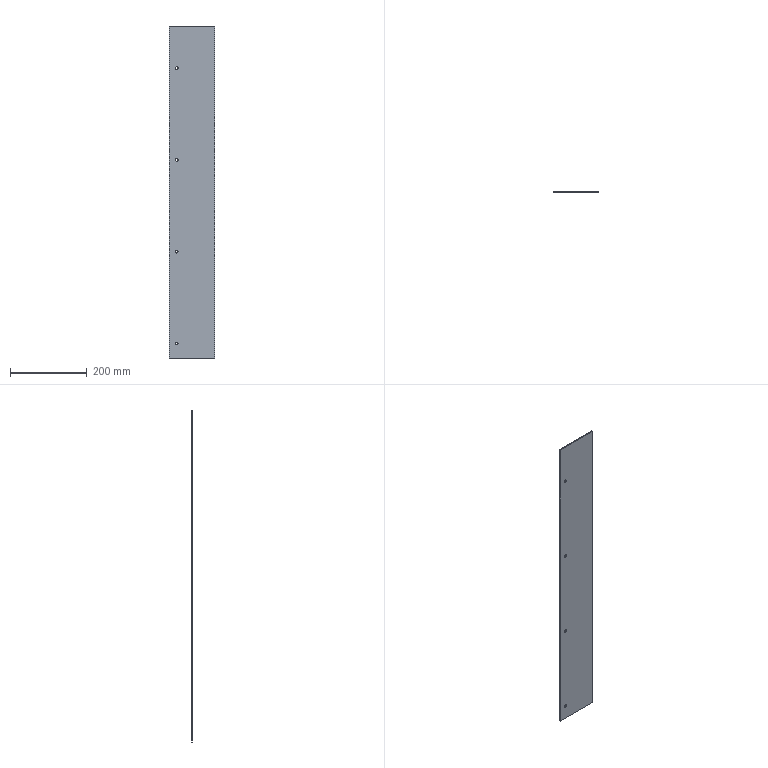Component | SolidWorks | 30-43A-1 | 1 solid | 14 faces | box 120 x 2 x 868 mm | volume 208012 mm3 | cylinder 8 | plane 6 | commonest cylinder face diameters 7 x8
STEP:
#1=COLOUR_RGB('',0.7922,0.8196,0.9333);
#2=FILL_AREA_STYLE_COLOUR('',#1);
#3=FILL_AREA_STYLE('',(#2));
#4=SURFACE_STYLE_FILL_AREA(#3);
#5=SURFACE_SIDE_STYLE('',(#4));
#6=SURFACE_STYLE_USAGE(.BOTH.,#5);
#7=PRESENTATION_STYLE_ASSIGNMENT((#6));
#8=CARTESIAN_POINT('',(-16.828,28.038,-30.965));
#9=VERTEX_POINT('',#8);
#10=CARTESIAN_POINT('',(-16.828,28.038,-31.24));
#11=VERTEX_POINT('',#10);
#12=CARTESIAN_POINT('',(-16.828,28.038,-31.102));
#13=DIRECTION('',(-0.,-1.,-0.));
#14=DIRECTION('',(0.,0.,-1.));
#15=AXIS2_PLACEMENT_3D('',#12,#13,#14);
#16=CIRCLE('',#15,0.1378);
#17=EDGE_CURVE('',#9,#11,#16,.T.);
#18=ORIENTED_EDGE('',*,*,#17,.T.);
#19=CARTESIAN_POINT('',(-16.828,28.116,-31.24));
#20=VERTEX_POINT('',#19);
#21=CARTESIAN_POINT('',(-16.828,27.723,-31.24));
#22=DIRECTION('',(0.,1.,0.));
#23=VECTOR('',#22,39.37);
#24=LINE('',#21,#23);
#25=EDGE_CURVE('',#11,#20,#24,.T.);
#26=ORIENTED_EDGE('',*,*,#25,.T.);
#27=CARTESIAN_POINT('',(-16.828,28.116,-30.965));
#28=VERTEX_POINT('',#27);
#29=CARTESIAN_POINT('',(-16.828,28.116,-31.102));
#30=DIRECTION('',(0.,1.,0.));
#31=DIRECTION('',(0.,0.,-1.));
#32=AXIS2_PLACEMENT_3D('',#29,#30,#31);
#33=CIRCLE('',#32,0.1378);
#34=EDGE_CURVE('',#20,#28,#33,.T.);
#35=ORIENTED_EDGE('',*,*,#34,.T.);
#36=CARTESIAN_POINT('',(-16.828,27.723,-30.965));
#37=DIRECTION('',(0.,1.,0.));
#38=VECTOR('',#37,39.37);
#39=LINE('',#36,#38);
#40=EDGE_CURVE('',#9,#28,#39,.T.);
#41=ORIENTED_EDGE('',*,*,#40,.F.);
#42=EDGE_LOOP('',(#18,#26,#35,#41));
#43=FACE_OUTER_BOUND('',#42,.T.);
#44=CARTESIAN_POINT('',(-16.828,27.723,-31.102));
#45=DIRECTION('',(0.,1.,0.));
#46=DIRECTION('',(0.,0.,1.));
#47=AXIS2_PLACEMENT_3D('',#44,#45,#46);
#48=CYLINDRICAL_SURFACE('',#47,0.1378);
#49=ADVANCED_FACE('',(#43),#48,.F.);
#50=CARTESIAN_POINT('',(-16.828,28.038,-21.516));
#51=VERTEX_POINT('',#50);
#52=CARTESIAN_POINT('',(-16.828,28.038,-21.791));
#53=VERTEX_POINT('',#52);
#54=CARTESIAN_POINT('',(-16.828,28.038,-21.654));
#55=DIRECTION('',(-0.,-1.,-0.));
#56=DIRECTION('',(0.,0.,-1.));
#57=AXIS2_PLACEMENT_3D('',#54,#55,#56);
#58=CIRCLE('',#57,0.1378);
#59=EDGE_CURVE('',#51,#53,#58,.T.);
#60=ORIENTED_EDGE('',*,*,#59,.T.);
#61=CARTESIAN_POINT('',(-16.828,28.116,-21.791));
#62=VERTEX_POINT('',#61);
#63=CARTESIAN_POINT('',(-16.828,27.723,-21.791));
#64=DIRECTION('',(0.,1.,0.));
#65=VECTOR('',#64,39.37);
#66=LINE('',#63,#65);
#67=EDGE_CURVE('',#53,#62,#66,.T.);
#68=ORIENTED_EDGE('',*,*,#67,.T.);
#69=CARTESIAN_POINT('',(-16.828,28.116,-21.516));
#70=VERTEX_POINT('',#69);
#71=CARTESIAN_POINT('',(-16.828,28.116,-21.654));
#72=DIRECTION('',(0.,1.,0.));
#73=DIRECTION('',(0.,0.,-1.));
#74=AXIS2_PLACEMENT_3D('',#71,#72,#73);
#75=CIRCLE('',#74,0.1378);
#76=EDGE_CURVE('',#62,#70,#75,.T.);
#77=ORIENTED_EDGE('',*,*,#76,.T.);
#78=CARTESIAN_POINT('',(-16.828,27.723,-21.516));
#79=DIRECTION('',(0.,1.,0.));
#80=VECTOR('',#79,39.37);
#81=LINE('',#78,#80);
#82=EDGE_CURVE('',#51,#70,#81,.T.);
#83=ORIENTED_EDGE('',*,*,#82,.F.);
#84=EDGE_LOOP('',(#60,#68,#77,#83));
#85=FACE_OUTER_BOUND('',#84,.T.);
#86=CARTESIAN_POINT('',(-16.828,27.723,-21.654));
#87=DIRECTION('',(0.,1.,0.));
#88=DIRECTION('',(0.,0.,1.));
#89=AXIS2_PLACEMENT_3D('',#86,#87,#88);
#90=CYLINDRICAL_SURFACE('',#89,0.1378);
#91=ADVANCED_FACE('',(#85),#90,.F.);
#92=CARTESIAN_POINT('',(-16.828,28.038,-12.067));
#93=VERTEX_POINT('',#92);
#94=CARTESIAN_POINT('',(-16.828,28.038,-12.343));
#95=VERTEX_POINT('',#94);
#96=CARTESIAN_POINT('',(-16.828,28.038,-12.205));
#97=DIRECTION('',(-0.,-1.,-0.));
#98=DIRECTION('',(0.,0.,-1.));
#99=AXIS2_PLACEMENT_3D('',#96,#97,#98);
#100=CIRCLE('',#99,0.1378);
#101=EDGE_CURVE('',#93,#95,#100,.T.);
#102=ORIENTED_EDGE('',*,*,#101,.T.);
#103=CARTESIAN_POINT('',(-16.828,28.116,-12.343));
#104=VERTEX_POINT('',#103);
#105=CARTESIAN_POINT('',(-16.828,27.723,-12.343));
#106=DIRECTION('',(0.,1.,0.));
#107=VECTOR('',#106,39.37);
#108=LINE('',#105,#107);
#109=EDGE_CURVE('',#95,#104,#108,.T.);
#110=ORIENTED_EDGE('',*,*,#109,.T.);
#111=CARTESIAN_POINT('',(-16.828,28.116,-12.067));
#112=VERTEX_POINT('',#111);
#113=CARTESIAN_POINT('',(-16.828,28.116,-12.205));
#114=DIRECTION('',(0.,1.,0.));
#115=DIRECTION('',(0.,0.,1.));
#116=AXIS2_PLACEMENT_3D('',#113,#114,#115);
#117=CIRCLE('',#116,0.1378);
#118=EDGE_CURVE('',#104,#112,#117,.T.);
#119=ORIENTED_EDGE('',*,*,#118,.T.);
#120=CARTESIAN_POINT('',(-16.828,27.723,-12.067));
#121=DIRECTION('',(0.,1.,0.));
#122=VECTOR('',#121,39.37);
#123=LINE('',#120,#122);
#124=EDGE_CURVE('',#93,#112,#123,.T.);
#125=ORIENTED_EDGE('',*,*,#124,.F.);
#126=EDGE_LOOP('',(#102,#110,#119,#125));
#127=FACE_OUTER_BOUND('',#126,.T.);
#128=CARTESIAN_POINT('',(-16.828,27.723,-12.205));
#129=DIRECTION('',(0.,1.,0.));
#130=DIRECTION('',(0.,0.,1.));
#131=AXIS2_PLACEMENT_3D('',#128,#129,#130);
#132=CYLINDRICAL_SURFACE('',#131,0.1378);
#133=ADVANCED_FACE('',(#127),#132,.F.);
#134=CARTESIAN_POINT('',(-16.828,28.038,-2.618));
#135=VERTEX_POINT('',#134);
#136=CARTESIAN_POINT('',(-16.828,28.038,-2.894));
#137=VERTEX_POINT('',#136);
#138=CARTESIAN_POINT('',(-16.828,28.038,-2.756));
#139=DIRECTION('',(-0.,-1.,-0.));
#140=DIRECTION('',(0.,0.,-1.));
#141=AXIS2_PLACEMENT_3D('',#138,#139,#140);
#142=CIRCLE('',#141,0.1378);
#143=EDGE_CURVE('',#135,#137,#142,.T.);
#144=ORIENTED_EDGE('',*,*,#143,.T.);
#145=CARTESIAN_POINT('',(-16.828,28.116,-2.894));
#146=VERTEX_POINT('',#145);
#147=CARTESIAN_POINT('',(-16.828,27.723,-2.894));
#148=DIRECTION('',(0.,1.,0.));
#149=VECTOR('',#148,39.37);
#150=LINE('',#147,#149);
#151=EDGE_CURVE('',#137,#146,#150,.T.);
#152=ORIENTED_EDGE('',*,*,#151,.T.);
#153=CARTESIAN_POINT('',(-16.828,28.116,-2.618));
#154=VERTEX_POINT('',#153);
#155=CARTESIAN_POINT('',(-16.828,28.116,-2.756));
#156=DIRECTION('',(0.,1.,0.));
#157=DIRECTION('',(0.,0.,1.));
#158=AXIS2_PLACEMENT_3D('',#155,#156,#157);
#159=CIRCLE('',#158,0.1378);
#160=EDGE_CURVE('',#146,#154,#159,.T.);
#161=ORIENTED_EDGE('',*,*,#160,.T.);
#162=CARTESIAN_POINT('',(-16.828,27.723,-2.618));
#163=DIRECTION('',(0.,1.,0.));
#164=VECTOR('',#163,39.37);
#165=LINE('',#162,#164);
#166=EDGE_CURVE('',#135,#154,#165,.T.);
#167=ORIENTED_EDGE('',*,*,#166,.F.);
#168=EDGE_LOOP('',(#144,#152,#161,#167));
#169=FACE_OUTER_BOUND('',#168,.T.);
#170=CARTESIAN_POINT('',(-16.828,27.723,-2.756));
#171=DIRECTION('',(0.,1.,0.));
#172=DIRECTION('',(0.,0.,1.));
#173=AXIS2_PLACEMENT_3D('',#170,#171,#172);
#174=CYLINDRICAL_SURFACE('',#173,0.1378);
#175=ADVANCED_FACE('',(#169),#174,.F.);
#176=CARTESIAN_POINT('',(-12.891,28.116,1.575));
#177=VERTEX_POINT('',#176);
#178=CARTESIAN_POINT('',(-17.615,28.116,1.575));
#179=VERTEX_POINT('',#178);
#180=CARTESIAN_POINT('',(-12.891,28.116,1.575));
#181=DIRECTION('',(-1.,0.,0.));
#182=VECTOR('',#181,39.37);
#183=LINE('',#180,#182);
#184=EDGE_CURVE('',#177,#179,#183,.T.);
#185=ORIENTED_EDGE('',*,*,#184,.T.);
#186=CARTESIAN_POINT('',(-17.615,28.038,1.575));
#187=VERTEX_POINT('',#186);
#188=CARTESIAN_POINT('',(-17.615,28.038,1.575));
#189=DIRECTION('',(0.,1.,0.));
#190=VECTOR('',#189,39.37);
#191=LINE('',#188,#190);
#192=EDGE_CURVE('',#187,#179,#191,.T.);
#193=ORIENTED_EDGE('',*,*,#192,.F.);
#194=CARTESIAN_POINT('',(-12.891,28.038,1.575));
#195=VERTEX_POINT('',#194);
#196=CARTESIAN_POINT('',(-12.891,28.038,1.575));
#197=DIRECTION('',(-1.,0.,0.));
#198=VECTOR('',#197,39.37);
#199=LINE('',#196,#198);
#200=EDGE_CURVE('',#195,#187,#199,.T.);
#201=ORIENTED_EDGE('',*,*,#200,.F.);
#202=CARTESIAN_POINT('',(-12.891,28.038,1.575));
#203=DIRECTION('',(0.,1.,0.));
#204=VECTOR('',#203,39.37);
#205=LINE('',#202,#204);
#206=EDGE_CURVE('',#195,#177,#205,.T.);
#207=ORIENTED_EDGE('',*,*,#206,.T.);
#208=EDGE_LOOP('',(#185,#193,#201,#207));
#209=FACE_OUTER_BOUND('',#208,.T.);
#210=CARTESIAN_POINT('',(-12.891,28.038,1.575));
#211=DIRECTION('',(-0.,0.,-1.));
#212=DIRECTION('',(0.,1.,0.));
#213=AXIS2_PLACEMENT_3D('',#210,#211,#212);
#214=PLANE('',#213);
#215=ADVANCED_FACE('',(#209),#214,.F.);
#216=CARTESIAN_POINT('',(-17.615,28.116,-32.598));
#217=VERTEX_POINT('',#216);
#218=CARTESIAN_POINT('',(-17.615,28.116,1.575));
#219=DIRECTION('',(-0.,0.,-1.));
#220=VECTOR('',#219,39.37);
#221=LINE('',#218,#220);
#222=EDGE_CURVE('',#179,#217,#221,.T.);
#223=ORIENTED_EDGE('',*,*,#222,.T.);
#224=CARTESIAN_POINT('',(-17.615,28.038,-32.598));
#225=VERTEX_POINT('',#224);
#226=CARTESIAN_POINT('',(-17.615,28.038,-32.598));
#227=DIRECTION('',(0.,1.,0.));
#228=VECTOR('',#227,39.37);
#229=LINE('',#226,#228);
#230=EDGE_CURVE('',#225,#217,#229,.T.);
#231=ORIENTED_EDGE('',*,*,#230,.F.);
#232=CARTESIAN_POINT('',(-17.615,28.038,1.575));
#233=DIRECTION('',(-0.,0.,-1.));
#234=VECTOR('',#233,39.37);
#235=LINE('',#232,#234);
#236=EDGE_CURVE('',#187,#225,#235,.T.);
#237=ORIENTED_EDGE('',*,*,#236,.F.);
#238=ORIENTED_EDGE('',*,*,#192,.T.);
#239=EDGE_LOOP('',(#223,#231,#237,#238));
#240=FACE_OUTER_BOUND('',#239,.T.);
#241=CARTESIAN_POINT('',(-17.615,28.038,1.575));
#242=DIRECTION('',(1.,-0.,-0.));
#243=DIRECTION('',(-0.,-1.,-0.));
#244=AXIS2_PLACEMENT_3D('',#241,#242,#243);
#245=PLANE('',#244);
#246=ADVANCED_FACE('',(#240),#245,.F.);
#247=CARTESIAN_POINT('',(-12.891,28.116,-32.598));
#248=VERTEX_POINT('',#247);
#249=CARTESIAN_POINT('',(-12.891,28.116,-32.598));
#250=DIRECTION('',(1.,-0.,-0.));
#251=VECTOR('',#250,39.37);
#252=LINE('',#249,#251);
#253=EDGE_CURVE('',#217,#248,#252,.T.);
#254=ORIENTED_EDGE('',*,*,#253,.T.);
#255=CARTESIAN_POINT('',(-12.891,28.038,-32.598));
#256=VERTEX_POINT('',#255);
#257=CARTESIAN_POINT('',(-12.891,28.038,-32.598));
#258=DIRECTION('',(0.,1.,0.));
#259=VECTOR('',#258,39.37);
#260=LINE('',#257,#259);
#261=EDGE_CURVE('',#256,#248,#260,.T.);
#262=ORIENTED_EDGE('',*,*,#261,.F.);
#263=CARTESIAN_POINT('',(-12.891,28.038,-32.598));
#264=DIRECTION('',(1.,-0.,-0.));
#265=VECTOR('',#264,39.37);
#266=LINE('',#263,#265);
#267=EDGE_CURVE('',#225,#256,#266,.T.);
#268=ORIENTED_EDGE('',*,*,#267,.F.);
#269=ORIENTED_EDGE('',*,*,#230,.T.);
#270=EDGE_LOOP('',(#254,#262,#268,#269));
#271=FACE_OUTER_BOUND('',#270,.T.);
#272=CARTESIAN_POINT('',(-12.891,28.038,-32.598));
#273=DIRECTION('',(0.,-0.,1.));
#274=DIRECTION('',(-0.,-1.,-0.));
#275=AXIS2_PLACEMENT_3D('',#272,#273,#274);
#276=PLANE('',#275);
#277=ADVANCED_FACE('',(#271),#276,.F.);
#278=CARTESIAN_POINT('',(-12.891,28.116,1.575));
#279=DIRECTION('',(0.,-0.,1.));
#280=VECTOR('',#279,39.37);
#281=LINE('',#278,#280);
#282=EDGE_CURVE('',#248,#177,#281,.T.);
#283=ORIENTED_EDGE('',*,*,#282,.T.);
#284=ORIENTED_EDGE('',*,*,#206,.F.);
#285=CARTESIAN_POINT('',(-12.891,28.038,1.575));
#286=DIRECTION('',(0.,-0.,1.));
#287=VECTOR('',#286,39.37);
#288=LINE('',#285,#287);
#289=EDGE_CURVE('',#256,#195,#288,.T.);
#290=ORIENTED_EDGE('',*,*,#289,.F.);
#291=ORIENTED_EDGE('',*,*,#261,.T.);
#292=EDGE_LOOP('',(#283,#284,#290,#291));
#293=FACE_OUTER_BOUND('',#292,.T.);
#294=CARTESIAN_POINT('',(-12.891,28.038,1.575));
#295=DIRECTION('',(-1.,0.,0.));
#296=DIRECTION('',(0.,1.,0.));
#297=AXIS2_PLACEMENT_3D('',#294,#295,#296);
#298=PLANE('',#297);
#299=ADVANCED_FACE('',(#293),#298,.F.);
#300=ORIENTED_EDGE('',*,*,#17,.F.);
#301=CARTESIAN_POINT('',(-16.828,28.038,-31.102));
#302=DIRECTION('',(-0.,-1.,-0.));
#303=DIRECTION('',(0.,0.,-1.));
#304=AXIS2_PLACEMENT_3D('',#301,#302,#303);
#305=CIRCLE('',#304,0.1378);
#306=EDGE_CURVE('',#11,#9,#305,.T.);
#307=ORIENTED_EDGE('',*,*,#306,.F.);
#308=EDGE_LOOP('',(#300,#307));
#309=FACE_BOUND('',#308,.T.);
#310=ORIENTED_EDGE('',*,*,#59,.F.);
#311=CARTESIAN_POINT('',(-16.828,28.038,-21.654));
#312=DIRECTION('',(-0.,-1.,-0.));
#313=DIRECTION('',(0.,0.,-1.));
#314=AXIS2_PLACEMENT_3D('',#311,#312,#313);
#315=CIRCLE('',#314,0.1378);
#316=EDGE_CURVE('',#53,#51,#315,.T.);
#317=ORIENTED_EDGE('',*,*,#316,.F.);
#318=EDGE_LOOP('',(#310,#317));
#319=FACE_BOUND('',#318,.T.);
#320=ORIENTED_EDGE('',*,*,#101,.F.);
#321=CARTESIAN_POINT('',(-16.828,28.038,-12.205));
#322=DIRECTION('',(-0.,-1.,-0.));
#323=DIRECTION('',(0.,0.,-1.));
#324=AXIS2_PLACEMENT_3D('',#321,#322,#323);
#325=CIRCLE('',#324,0.1378);
#326=EDGE_CURVE('',#95,#93,#325,.T.);
#327=ORIENTED_EDGE('',*,*,#326,.F.);
#328=EDGE_LOOP('',(#320,#327));
#329=FACE_BOUND('',#328,.T.);
#330=ORIENTED_EDGE('',*,*,#143,.F.);
#331=CARTESIAN_POINT('',(-16.828,28.038,-2.756));
#332=DIRECTION('',(-0.,-1.,-0.));
#333=DIRECTION('',(0.,0.,-1.));
#334=AXIS2_PLACEMENT_3D('',#331,#332,#333);
#335=CIRCLE('',#334,0.1378);
#336=EDGE_CURVE('',#137,#135,#335,.T.);
#337=ORIENTED_EDGE('',*,*,#336,.F.);
#338=EDGE_LOOP('',(#330,#337));
#339=FACE_BOUND('',#338,.T.);
#340=ORIENTED_EDGE('',*,*,#200,.T.);
#341=ORIENTED_EDGE('',*,*,#236,.T.);
#342=ORIENTED_EDGE('',*,*,#267,.T.);
#343=ORIENTED_EDGE('',*,*,#289,.T.);
#344=EDGE_LOOP('',(#340,#341,#342,#343));
#345=FACE_OUTER_BOUND('',#344,.T.);
#346=CARTESIAN_POINT('',(-17.615,28.038,1.575));
#347=DIRECTION('',(-0.,-1.,-0.));
#348=DIRECTION('',(-0.,0.,-1.));
#349=AXIS2_PLACEMENT_3D('',#346,#347,#348);
#350=PLANE('',#349);
#351=ADVANCED_FACE('',(#309,#319,#329,#339,#345),#350,.T.);
#352=CARTESIAN_POINT('',(-16.828,28.116,-31.102));
#353=DIRECTION('',(0.,1.,0.));
#354=DIRECTION('',(0.,0.,-1.));
#355=AXIS2_PLACEMENT_3D('',#352,#353,#354);
#356=CIRCLE('',#355,0.1378);
#357=EDGE_CURVE('',#28,#20,#356,.T.);
#358=ORIENTED_EDGE('',*,*,#357,.F.);
#359=ORIENTED_EDGE('',*,*,#34,.F.);
#360=EDGE_LOOP('',(#358,#359));
#361=FACE_BOUND('',#360,.T.);
#362=CARTESIAN_POINT('',(-16.828,28.116,-21.654));
#363=DIRECTION('',(0.,1.,0.));
#364=DIRECTION('',(0.,0.,-1.));
#365=AXIS2_PLACEMENT_3D('',#362,#363,#364);
#366=CIRCLE('',#365,0.1378);
#367=EDGE_CURVE('',#70,#62,#366,.T.);
#368=ORIENTED_EDGE('',*,*,#367,.F.);
#369=ORIENTED_EDGE('',*,*,#76,.F.);
#370=EDGE_LOOP('',(#368,#369));
#371=FACE_BOUND('',#370,.T.);
#372=CARTESIAN_POINT('',(-16.828,28.116,-12.205));
#373=DIRECTION('',(0.,1.,0.));
#374=DIRECTION('',(0.,0.,1.));
#375=AXIS2_PLACEMENT_3D('',#372,#373,#374);
#376=CIRCLE('',#375,0.1378);
#377=EDGE_CURVE('',#112,#104,#376,.T.);
#378=ORIENTED_EDGE('',*,*,#377,.F.);
#379=ORIENTED_EDGE('',*,*,#118,.F.);
#380=EDGE_LOOP('',(#378,#379));
#381=FACE_BOUND('',#380,.T.);
#382=CARTESIAN_POINT('',(-16.828,28.116,-2.756));
#383=DIRECTION('',(0.,1.,0.));
#384=DIRECTION('',(0.,0.,1.));
#385=AXIS2_PLACEMENT_3D('',#382,#383,#384);
#386=CIRCLE('',#385,0.1378);
#387=EDGE_CURVE('',#154,#146,#386,.T.);
#388=ORIENTED_EDGE('',*,*,#387,.F.);
#389=ORIENTED_EDGE('',*,*,#160,.F.);
#390=EDGE_LOOP('',(#388,#389));
#391=FACE_BOUND('',#390,.T.);
#392=ORIENTED_EDGE('',*,*,#184,.F.);
#393=ORIENTED_EDGE('',*,*,#282,.F.);
#394=ORIENTED_EDGE('',*,*,#253,.F.);
#395=ORIENTED_EDGE('',*,*,#222,.F.);
#396=EDGE_LOOP('',(#392,#393,#394,#395));
#397=FACE_OUTER_BOUND('',#396,.T.);
#398=CARTESIAN_POINT('',(-17.615,28.116,1.575));
#399=DIRECTION('',(-0.,-1.,-0.));
#400=DIRECTION('',(-0.,0.,-1.));
#401=AXIS2_PLACEMENT_3D('',#398,#399,#400);
#402=PLANE('',#401);
#403=ADVANCED_FACE('',(#361,#371,#381,#391,#397),#402,.F.);
#404=ORIENTED_EDGE('',*,*,#151,.F.);
#405=ORIENTED_EDGE('',*,*,#336,.T.);
#406=ORIENTED_EDGE('',*,*,#166,.T.);
#407=ORIENTED_EDGE('',*,*,#387,.T.);
#408=EDGE_LOOP('',(#404,#405,#406,#407));
#409=FACE_OUTER_BOUND('',#408,.T.);
#410=CARTESIAN_POINT('',(-16.828,27.723,-2.756));
#411=DIRECTION('',(0.,1.,0.));
#412=DIRECTION('',(0.,0.,1.));
#413=AXIS2_PLACEMENT_3D('',#410,#411,#412);
#414=CYLINDRICAL_SURFACE('',#413,0.1378);
#415=ADVANCED_FACE('',(#409),#414,.F.);
#416=ORIENTED_EDGE('',*,*,#109,.F.);
#417=ORIENTED_EDGE('',*,*,#326,.T.);
#418=ORIENTED_EDGE('',*,*,#124,.T.);
#419=ORIENTED_EDGE('',*,*,#377,.T.);
#420=EDGE_LOOP('',(#416,#417,#418,#419));
#421=FACE_OUTER_BOUND('',#420,.T.);
#422=CARTESIAN_POINT('',(-16.828,27.723,-12.205));
#423=DIRECTION('',(0.,1.,0.));
#424=DIRECTION('',(0.,0.,1.));
#425=AXIS2_PLACEMENT_3D('',#422,#423,#424);
#426=CYLINDRICAL_SURFACE('',#425,0.1378);
#427=ADVANCED_FACE('',(#421),#426,.F.);
#428=ORIENTED_EDGE('',*,*,#67,.F.);
#429=ORIENTED_EDGE('',*,*,#316,.T.);
#430=ORIENTED_EDGE('',*,*,#82,.T.);
#431=ORIENTED_EDGE('',*,*,#367,.T.);
#432=EDGE_LOOP('',(#428,#429,#430,#431));
#433=FACE_OUTER_BOUND('',#432,.T.);
#434=CARTESIAN_POINT('',(-16.828,27.723,-21.654));
#435=DIRECTION('',(0.,1.,0.));
#436=DIRECTION('',(0.,0.,1.));
#437=AXIS2_PLACEMENT_3D('',#434,#435,#436);
#438=CYLINDRICAL_SURFACE('',#437,0.1378);
#439=ADVANCED_FACE('',(#433),#438,.F.);
#440=ORIENTED_EDGE('',*,*,#25,.F.);
#441=ORIENTED_EDGE('',*,*,#306,.T.);
#442=ORIENTED_EDGE('',*,*,#40,.T.);
#443=ORIENTED_EDGE('',*,*,#357,.T.);
#444=EDGE_LOOP('',(#440,#441,#442,#443));
#445=FACE_OUTER_BOUND('',#444,.T.);
#446=CARTESIAN_POINT('',(-16.828,27.723,-31.102));
#447=DIRECTION('',(0.,1.,0.));
#448=DIRECTION('',(0.,0.,1.));
#449=AXIS2_PLACEMENT_3D('',#446,#447,#448);
#450=CYLINDRICAL_SURFACE('',#449,0.1378);
#451=ADVANCED_FACE('',(#445),#450,.F.);
#452=CLOSED_SHELL('',(#49,#91,#133,#175,#215,#246,#277,#299,#351,#403,#415,#427,#439,#451));
#453=MANIFOLD_SOLID_BREP('',#452);
#454=STYLED_ITEM('',(#7),#453);
#455=PRESENTATION_LAYER_ASSIGNMENT('','',(#454));
#456=(LENGTH_UNIT()NAMED_UNIT(*)SI_UNIT($,.METRE.));
#457=LENGTH_MEASURE_WITH_UNIT(LENGTH_MEASURE(0.0254),#456);
#458=DIMENSIONAL_EXPONENTS(1.,0.,0.,0.,0.,0.,0.);
#459=(CONVERSION_BASED_UNIT('',#457)LENGTH_UNIT()NAMED_UNIT(#458));
#460=UNCERTAINTY_MEASURE_WITH_UNIT(LENGTH_MEASURE(0.00001),#459,'','');
#461=(NAMED_UNIT(*)PLANE_ANGLE_UNIT()SI_UNIT($,.RADIAN.));
#462=(NAMED_UNIT(*)SI_UNIT($,.STERADIAN.)SOLID_ANGLE_UNIT());
#463=(GEOMETRIC_REPRESENTATION_CONTEXT(3)GLOBAL_UNCERTAINTY_ASSIGNED_CONTEXT((#460))GLOBAL_UNIT_ASSIGNED_CONTEXT((#459,#461,#462))REPRESENTATION_CONTEXT('',''));
#464=MECHANICAL_DESIGN_GEOMETRIC_PRESENTATION_REPRESENTATION('',(#454),#463);
#465=CARTESIAN_POINT('',(0.,0.,0.));
#466=DIRECTION('',(0.,0.,1.));
#467=DIRECTION('',(1.,0.,0.));
#468=AXIS2_PLACEMENT_3D('',#465,#466,#467);
#469=(LENGTH_UNIT()NAMED_UNIT(*)SI_UNIT($,.METRE.));
#470=LENGTH_MEASURE_WITH_UNIT(LENGTH_MEASURE(0.0254),#469);
#471=DIMENSIONAL_EXPONENTS(1.,0.,0.,0.,0.,0.,0.);
#472=(CONVERSION_BASED_UNIT('',#470)LENGTH_UNIT()NAMED_UNIT(#471));
#473=UNCERTAINTY_MEASURE_WITH_UNIT(LENGTH_MEASURE(0.00001),#472,'','');
#474=(NAMED_UNIT(*)PLANE_ANGLE_UNIT()SI_UNIT($,.RADIAN.));
#475=(NAMED_UNIT(*)SI_UNIT($,.STERADIAN.)SOLID_ANGLE_UNIT());
#476=(GEOMETRIC_REPRESENTATION_CONTEXT(3)GLOBAL_UNCERTAINTY_ASSIGNED_CONTEXT((#473))GLOBAL_UNIT_ASSIGNED_CONTEXT((#472,#474,#475))REPRESENTATION_CONTEXT('',''));
#477=ADVANCED_BREP_SHAPE_REPRESENTATION('',(#453,#468),#476);